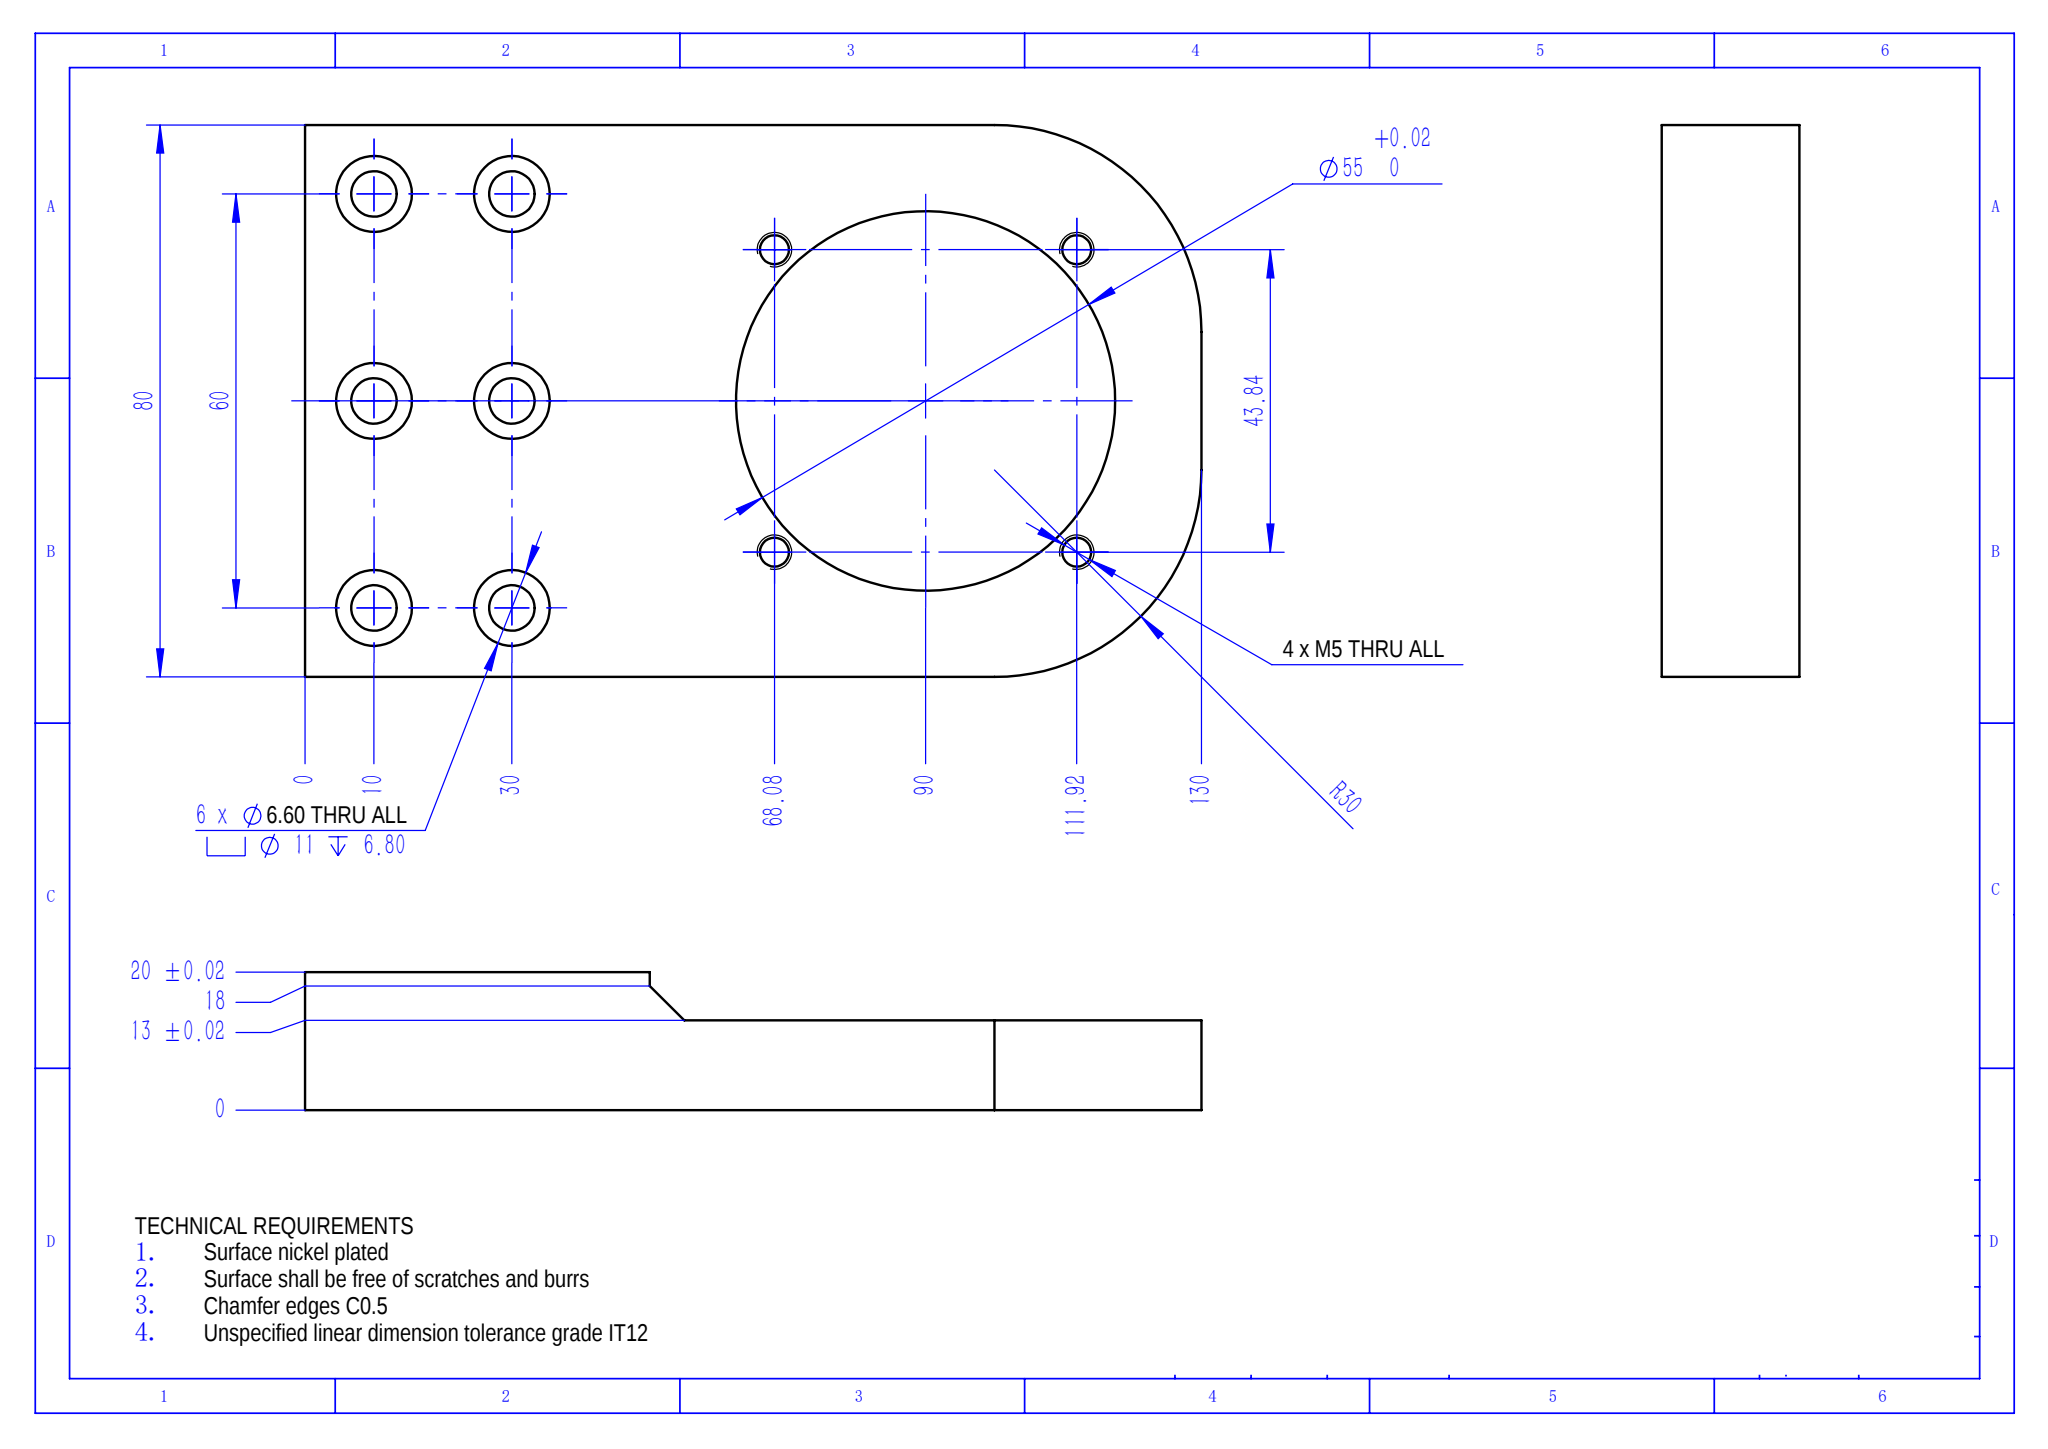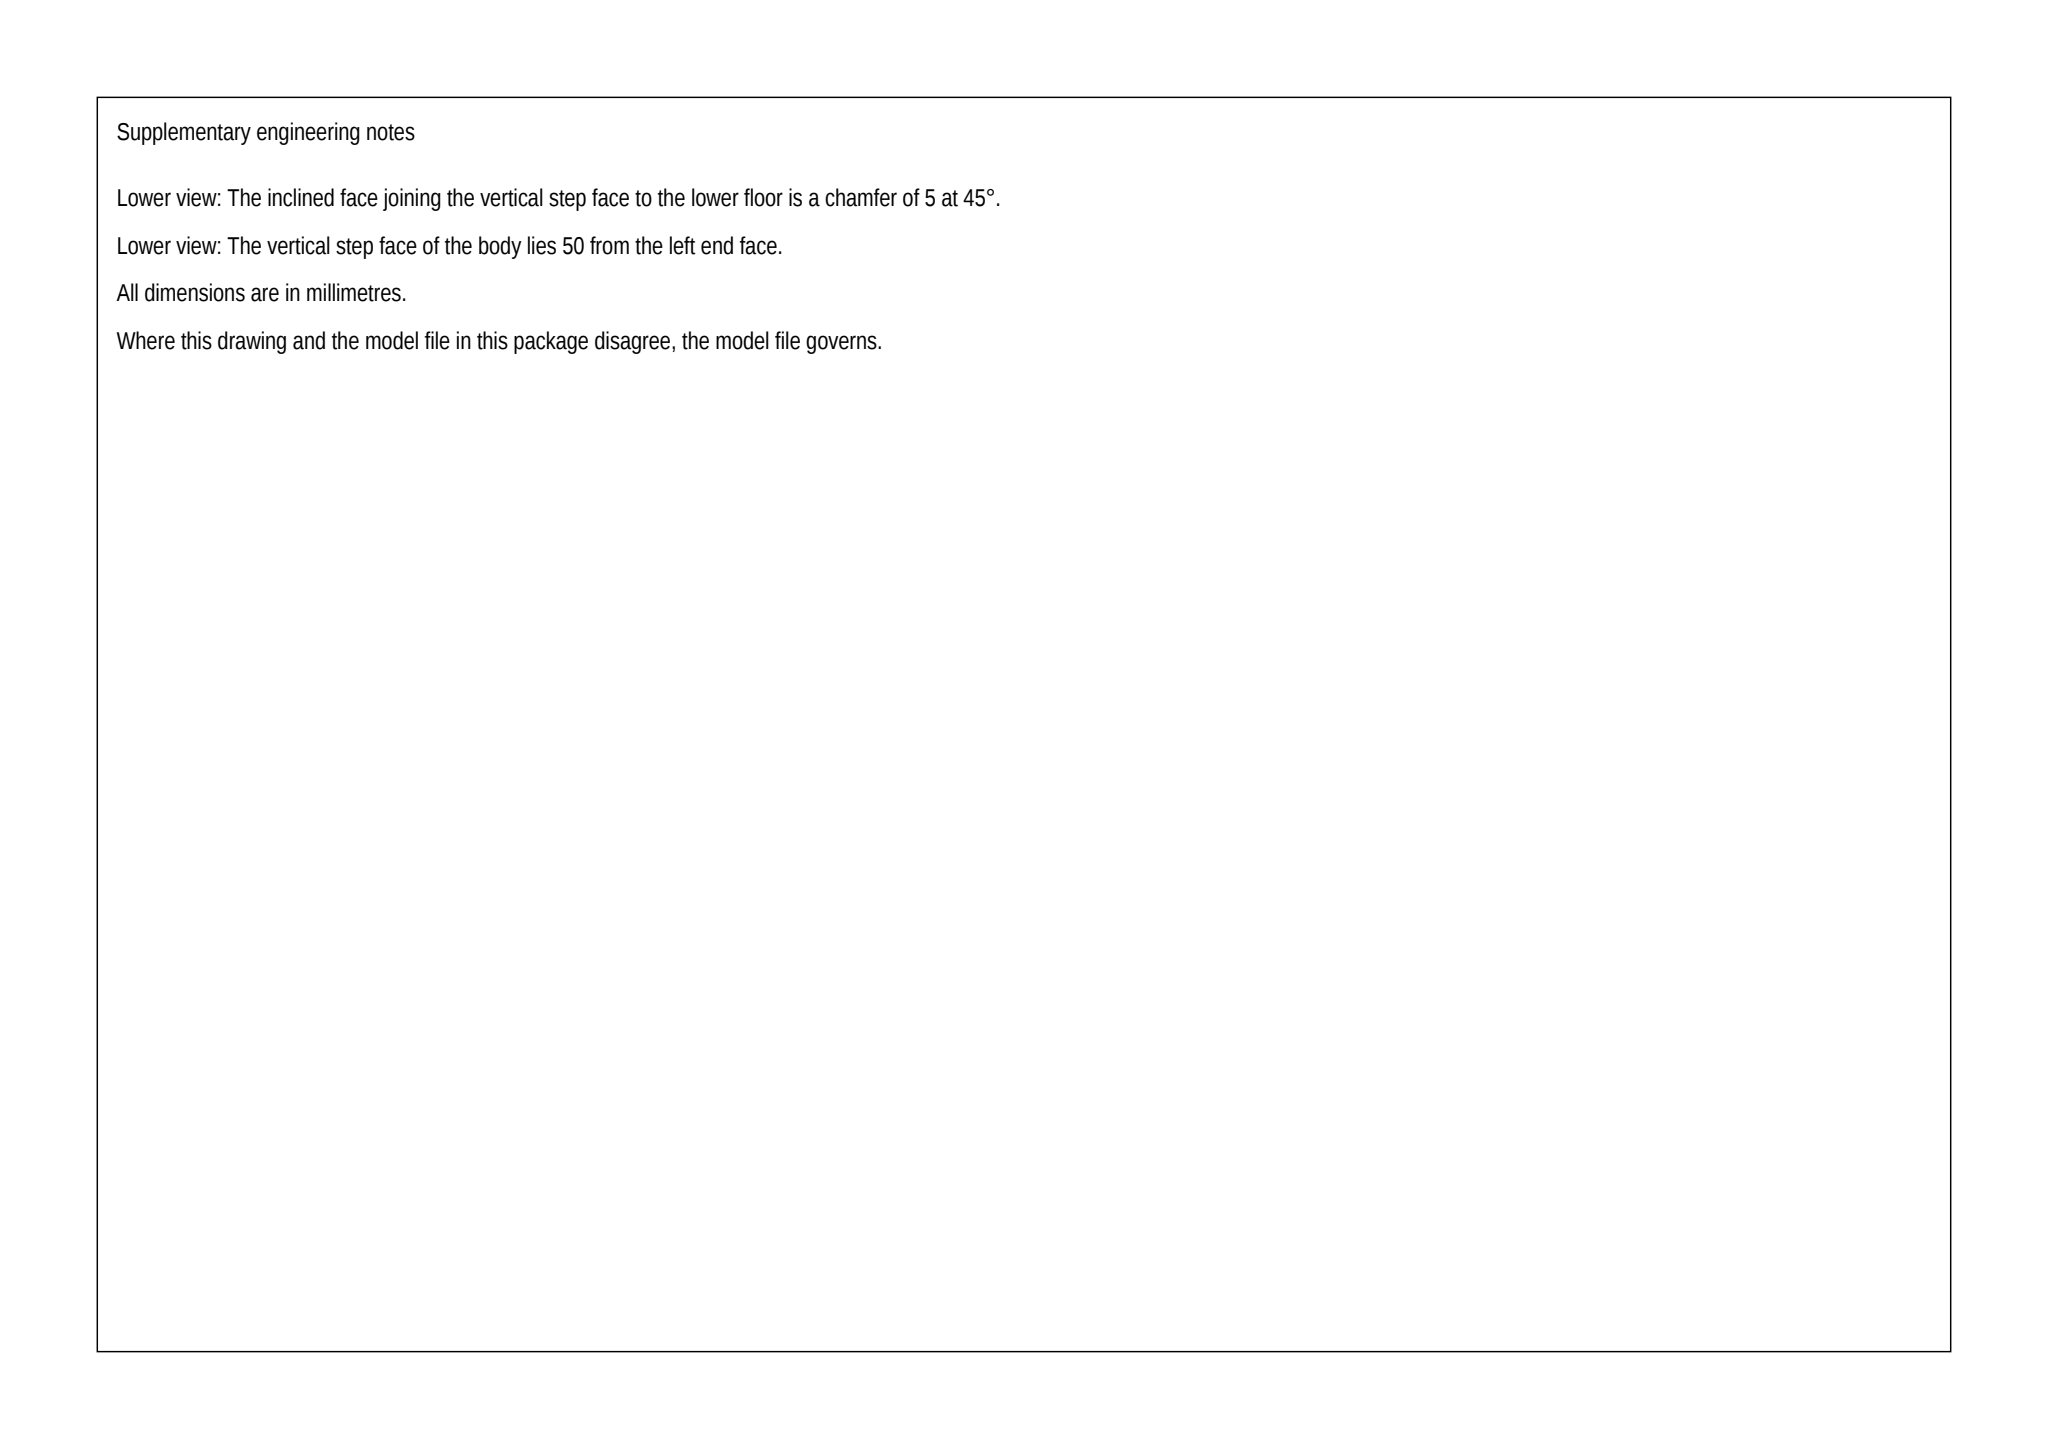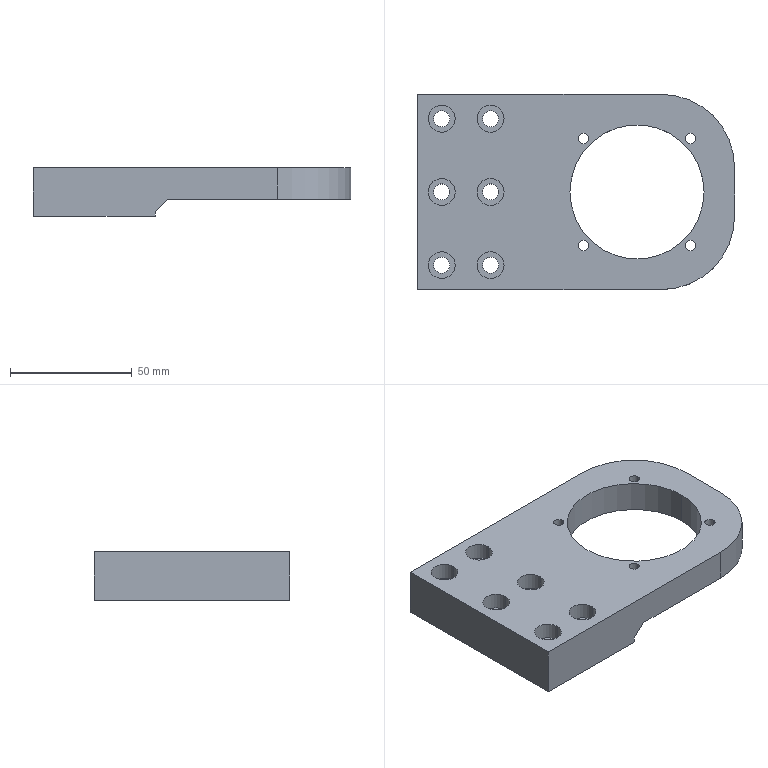Part | SolidWorks | mm | 1 solid | 51 faces | box 130 x 80 x 20 mm | volume 120985 mm3 | cylinder 36 | plane 15 | commonest cylinder face diameters 11 x12 6.6 x12 4.2 x8 55 x2 60 x2
build123d program:
from build123d import *

# Parameters (mm, degrees)
SKETCH1_W                                         = 130
SKETCH1_H                                         = 80
SKETCH1_R                                         = 27.5
BOSS_EXTRUDE1_DEPTH                               = 10
M5_TAPPED_HOLE1_D                                 = 4.2
HOLE_SIZE_ACCORDING_TO_HEXAGON_SOCKET_D           = 6.6
HOLE_SIZE_ACCORDING_TO_HEXAGON_SOCKET_CBORE_D     = 11
HOLE_SIZE_ACCORDING_TO_HEXAGON_SOCKET_CBORE_DEPTH = 6.8
SKETCH6_W                                         = 80
SKETCH6_H                                         = 80
CUT_EXTRUDE1_DEPTH                                = 7
CHAMFER2_SIZE                                     = 5
FILLET1_R                                         = 30


with BuildPart() as part:
    # Sketch1 → Boss-Extrude1 (new, symmetric)
    with BuildSketch(Plane.XY):
        with Locations((65, 0)):
            Rectangle(SKETCH1_W, SKETCH1_H)
        with Locations((90, 0)):
            Circle(SKETCH1_R, mode=Mode.SUBTRACT)
    extrude(amount=BOSS_EXTRUDE1_DEPTH, both=True)

    # M5 Tapped Hole1 (through all)
    with Locations(Plane.XY.offset(10)):
        with Locations((111.92, 21.92), (68.08, 21.92), (68.08, -21.92), (111.92, -21.92)):
            Hole(M5_TAPPED_HOLE1_D / 2)

    # Hole Size _ according to_ Hexagon Socket (through all)
    with Locations(Plane(origin=(0, 15, 10), x_dir=(1, 0, 0), z_dir=(0, 0, 1))):
        with Locations((30, -15), (10, -45), (30, -45), (10, 15), (30, 15), (10, -15)):
            CounterBoreHole(HOLE_SIZE_ACCORDING_TO_HEXAGON_SOCKET_D / 2, HOLE_SIZE_ACCORDING_TO_HEXAGON_SOCKET_CBORE_D / 2, HOLE_SIZE_ACCORDING_TO_HEXAGON_SOCKET_CBORE_DEPTH)

    # Sketch6 → Cut-Extrude1 (cut)
    with BuildSketch(Plane(origin=(0, 0, -10), x_dir=(-1, 0, 0), z_dir=(0, 0, -1))):
        with Locations((-90, 0)):
            Rectangle(SKETCH6_W, SKETCH6_H)
    extrude(amount=-CUT_EXTRUDE1_DEPTH, mode=Mode.SUBTRACT)

    # Chamfer2
    chamfer2_edges = [part.edges().sort_by_distance(p)[0] for p in [
        (50, 0, -3),
    ]]
    chamfer(chamfer2_edges, length=CHAMFER2_SIZE)

    # Fillet1
    fillet1_edges = [part.edges().sort_by_distance(p)[0] for p in [
        (130, 40, 3.5),
        (130, -40, 3.5),
    ]]
    fillet(fillet1_edges, radius=FILLET1_R)


solid = part.part